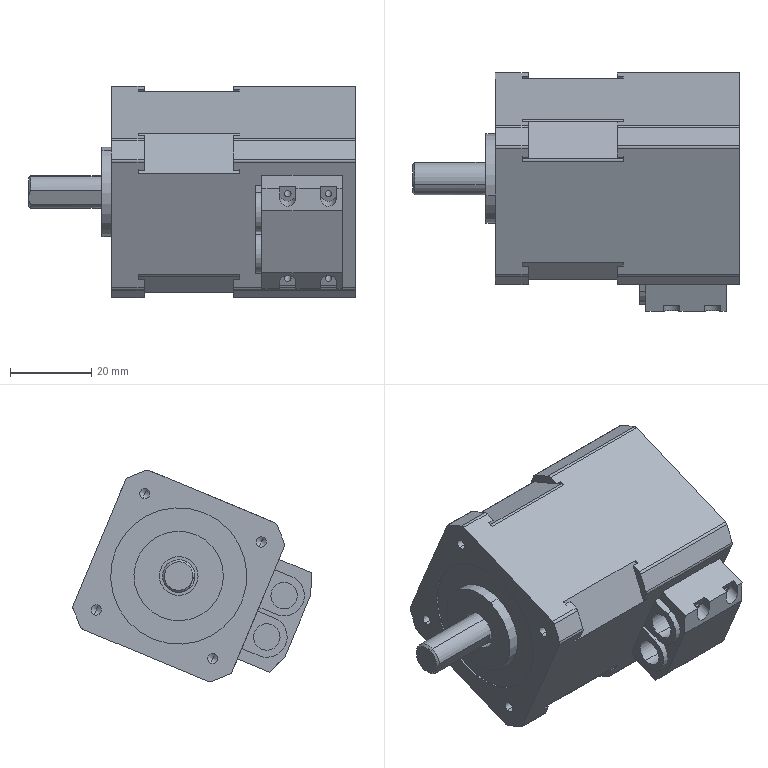Component | SolidWorks | 42mmHybridStepperMotor-1 | 1 solid | 162 faces | volume 109525 mm3 | plane 75 | cylinder 60 | cone 27 | commonest cylinder face diameters 2 x22 1.6 x8 2.5 x8 6.5 x4 3.2 x4 4 x4 8 x2 9.5 x2